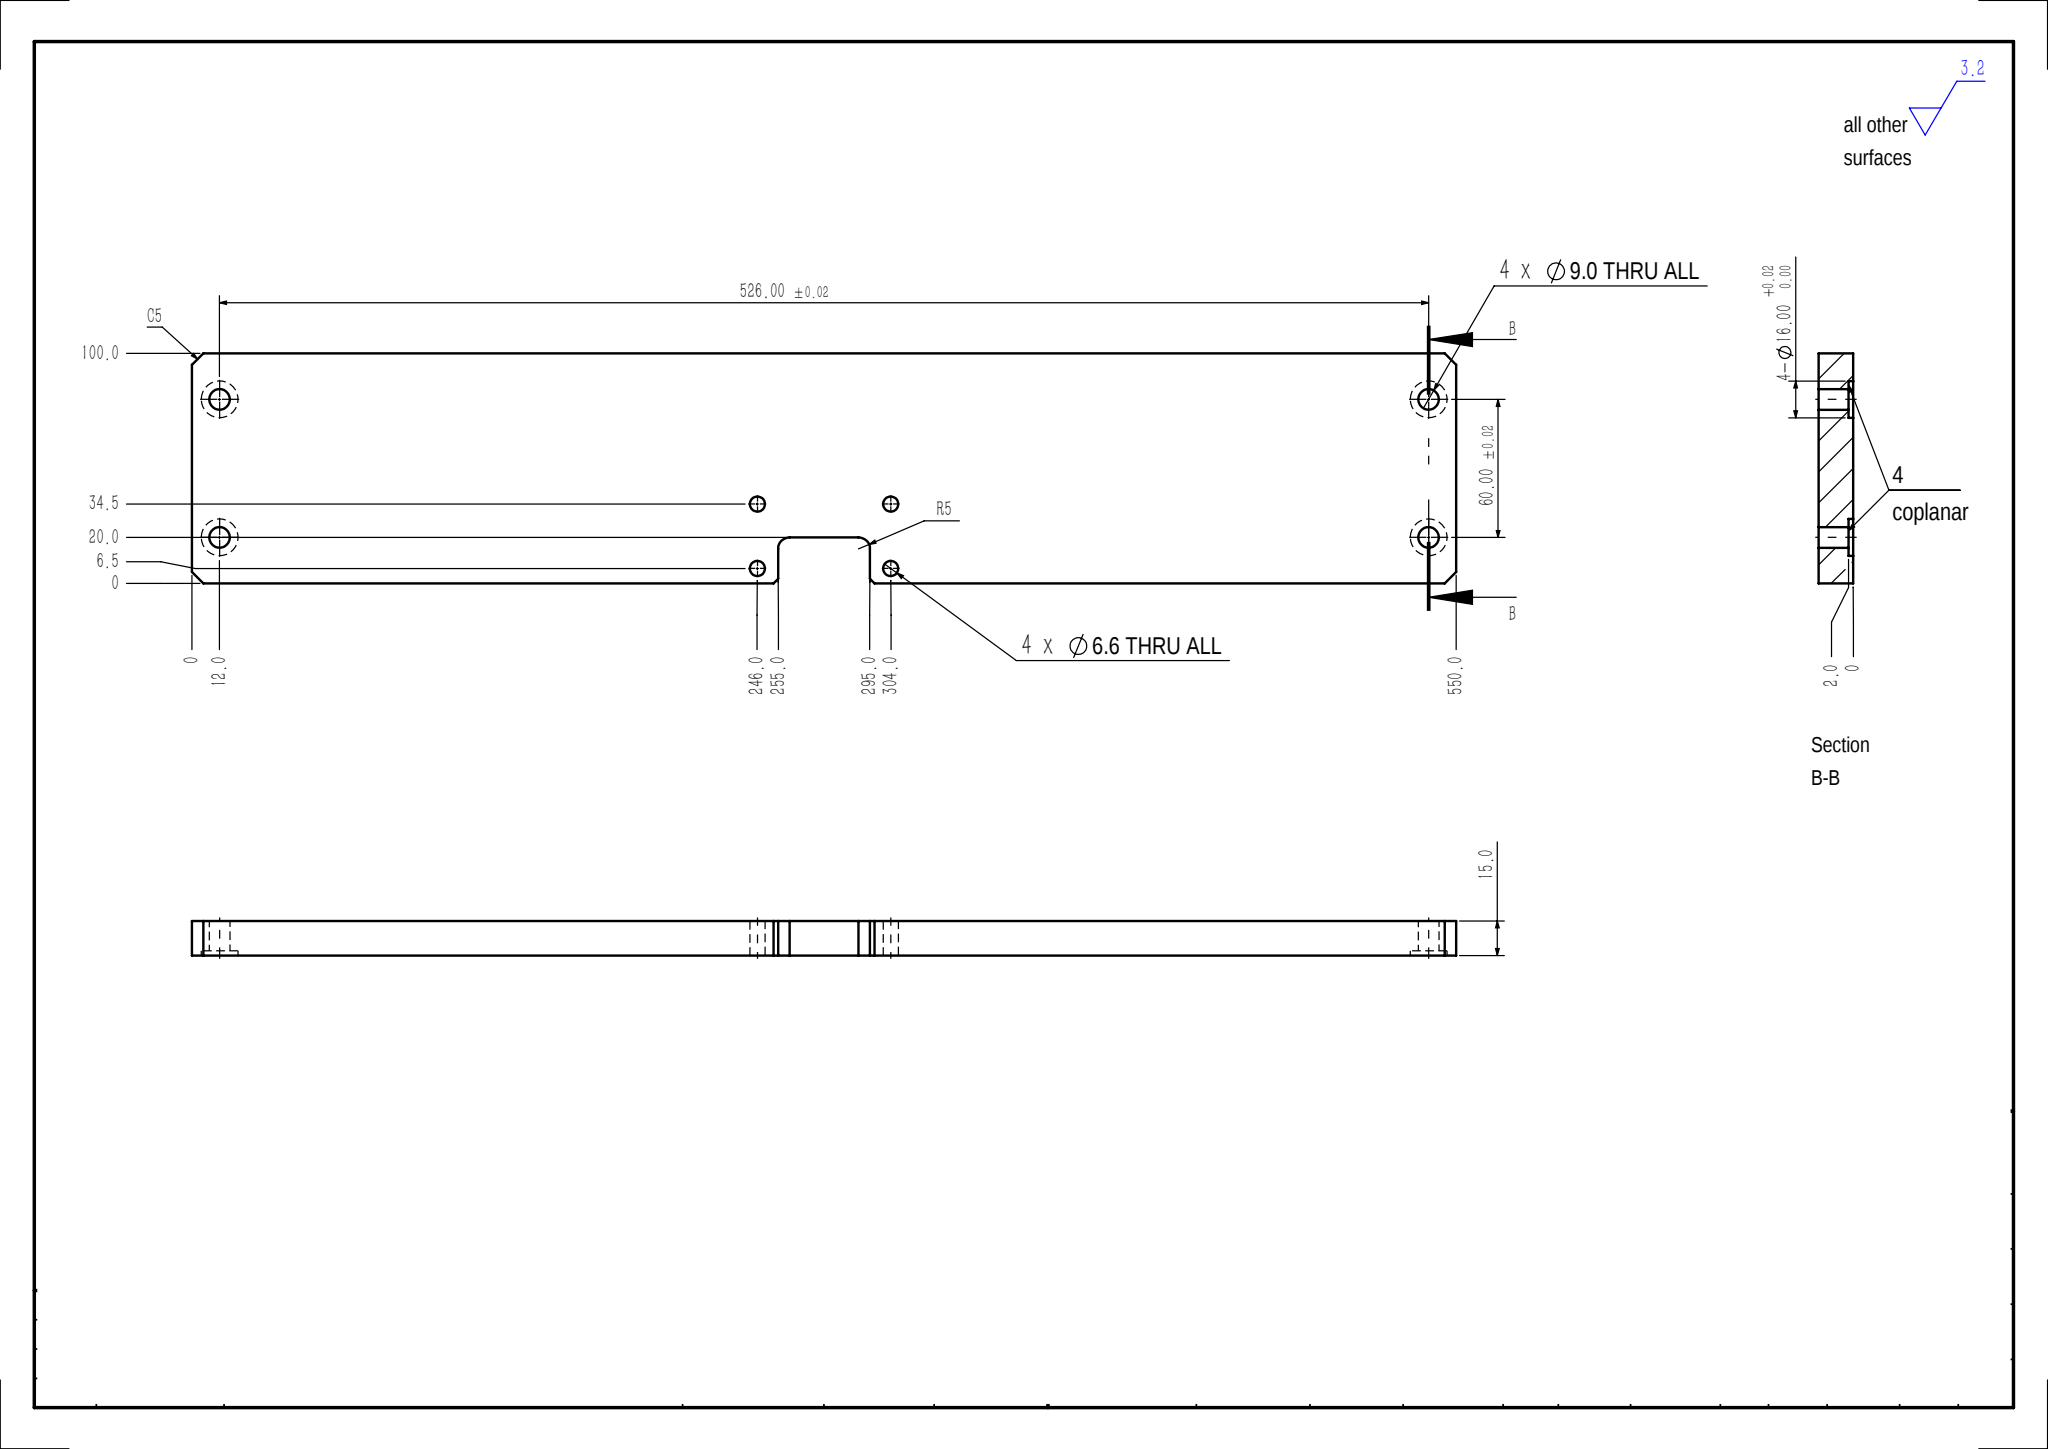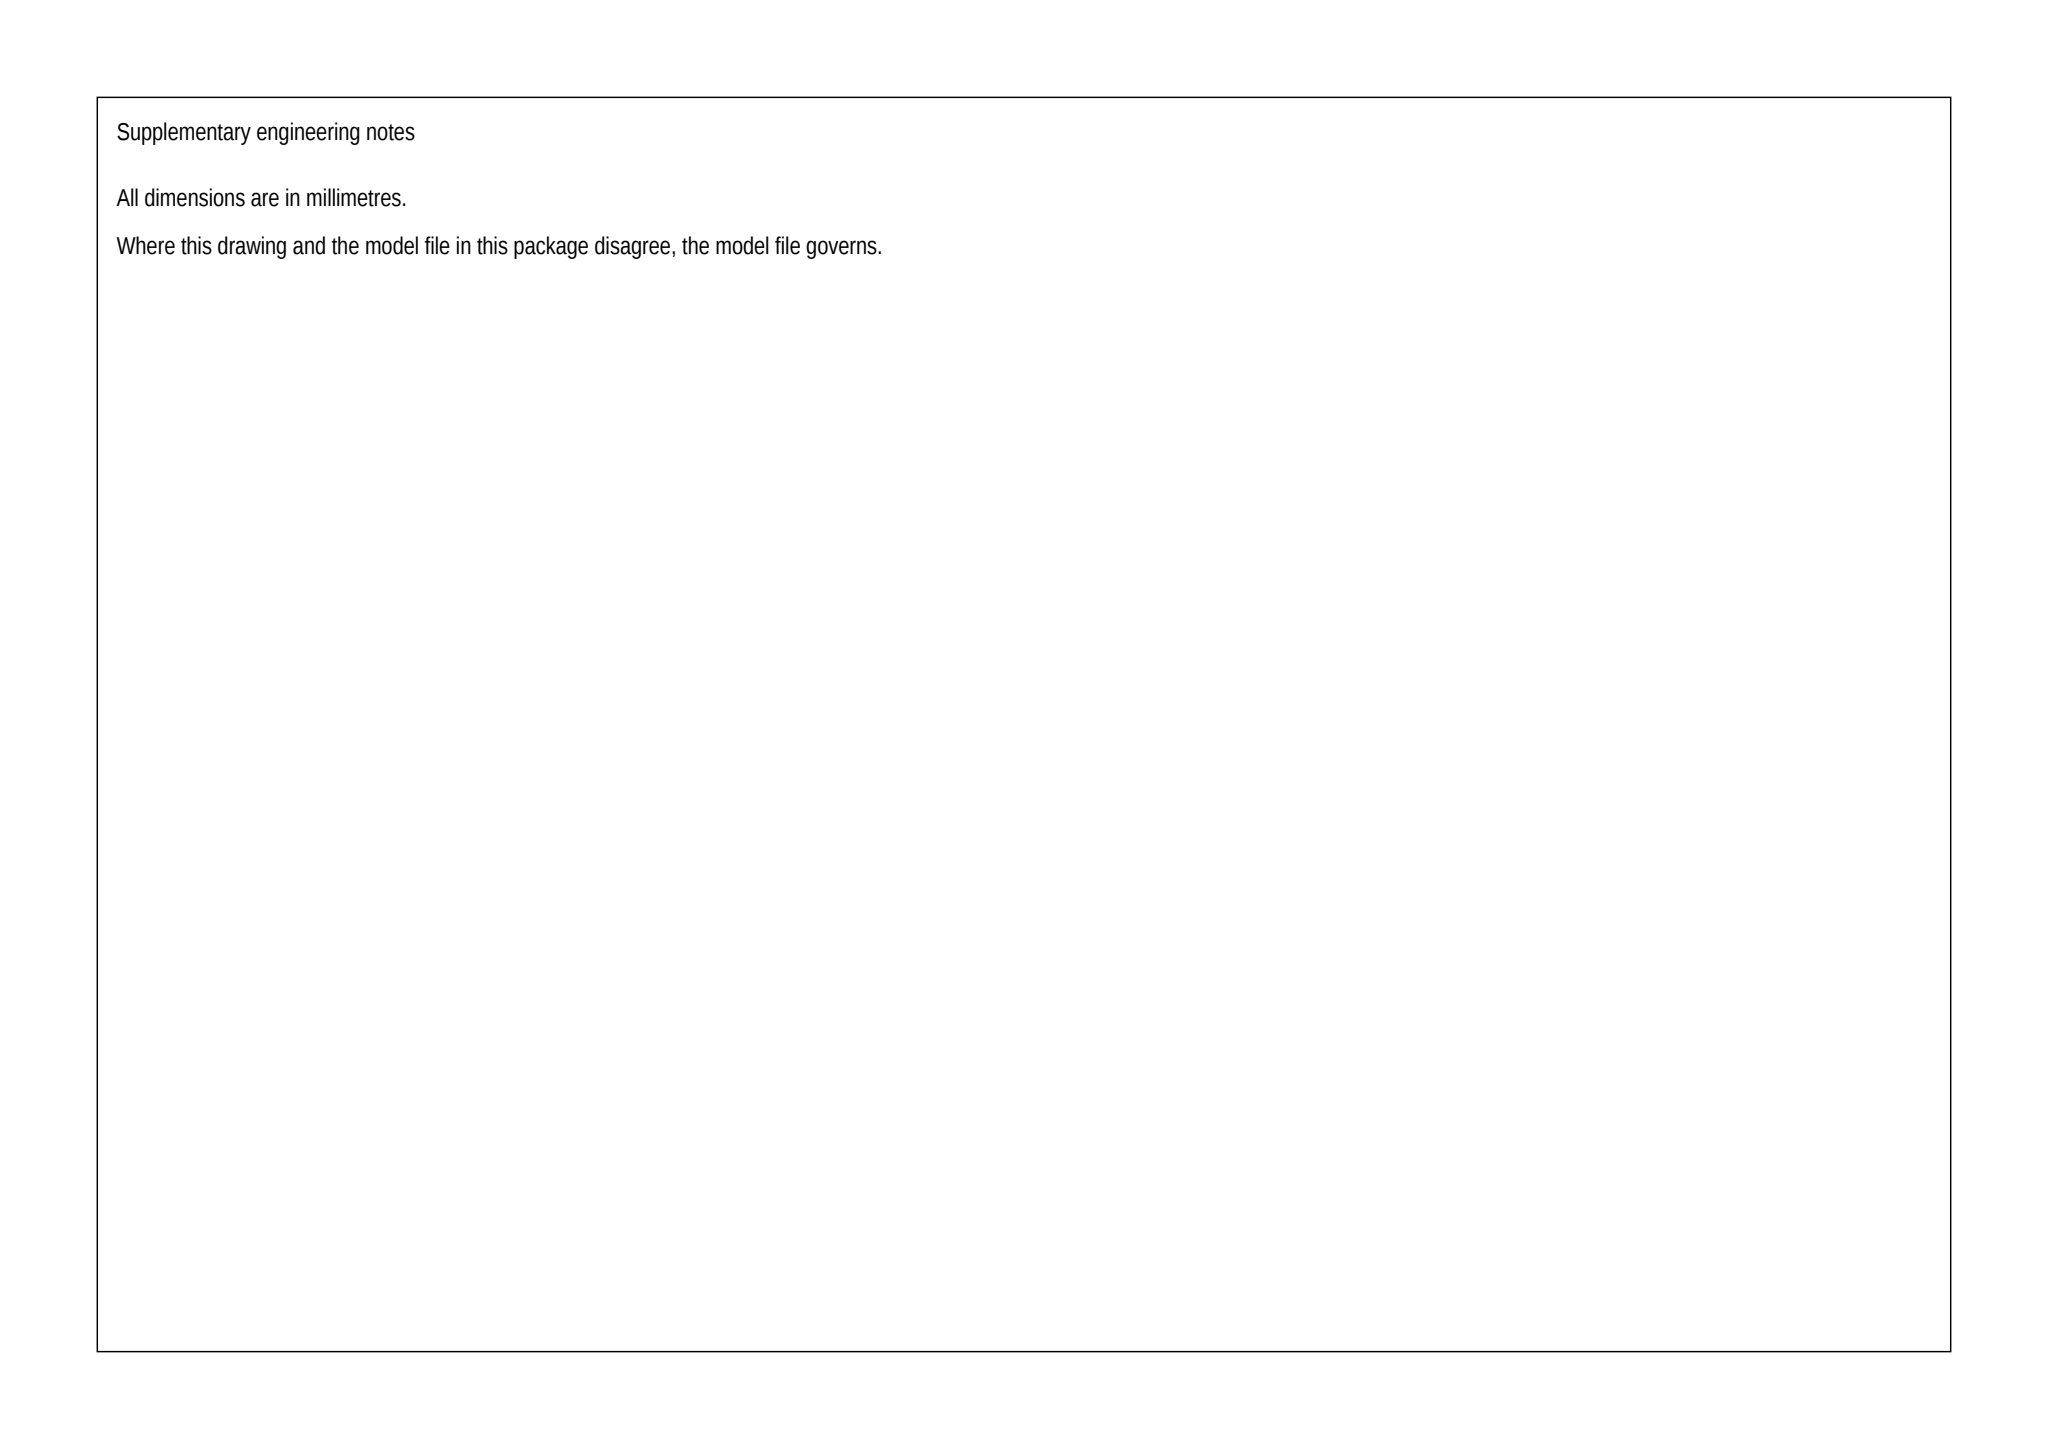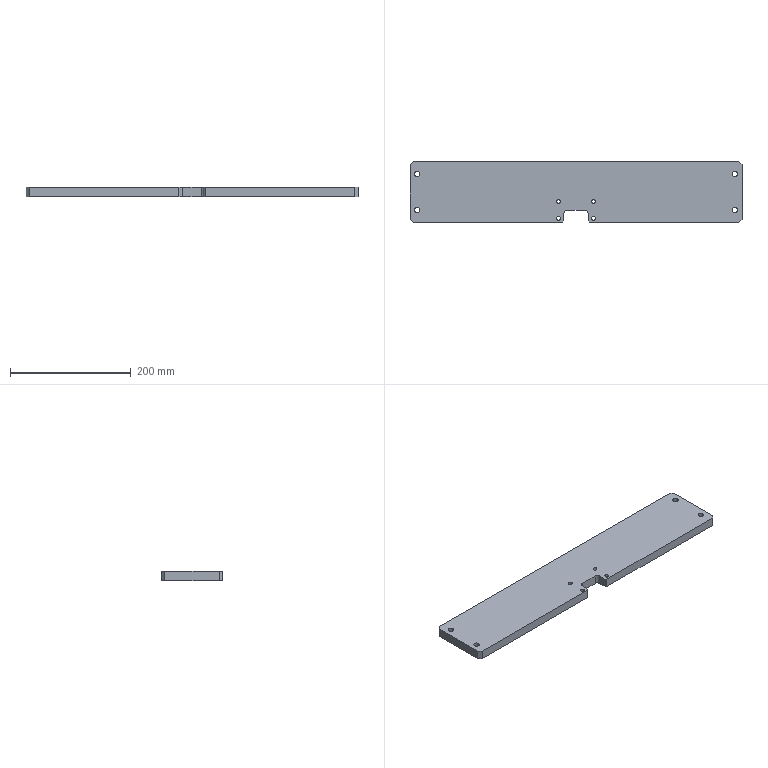Part | SolidWorks | mm | 1 solid | 46 faces | box 550 x 100 x 15 mm | volume 805382 mm3 | cylinder 26 | plane 20 | commonest cylinder face diameters 6.6 x8 16 x8 9 x8 10 x2
build123d program:
from build123d import *

# Parameters (mm, degrees)
SKETCH1_W             = 550
SKETCH1_H             = 100
BOSS_EXTRUDE1_DEPTH   = 15
M8_CLEARANCE_HOLE_1_D = 9
SKETCH5_R             = 8
CUT_EXTRUDE1_DEPTH    = 2
CHAMFER1_SIZE         = 5
SKETCH6_W             = 40
SKETCH6_H             = 20
CUT_EXTRUDE2_DEPTH    = 280.911
FILLET1_R             = 5
CHAMFER2_SIZE         = 2
M6_CLEARANCE_HOLE_1_D = 6.6


with BuildPart() as part:
    # Sketch1 → Boss-Extrude1 (new body)
    with BuildSketch(Plane.XY):
        Rectangle(SKETCH1_W, SKETCH1_H)
    extrude(amount=BOSS_EXTRUDE1_DEPTH)

    # M8 Clearance Hole 1 (through all)
    with Locations(Plane.XY.offset(15)):
        with Locations((-263, 30), (-263, -30), (263, -30), (263, 30)):
            Hole(M8_CLEARANCE_HOLE_1_D / 2)

    # Sketch5 → Cut-Extrude1 (cut)
    with BuildSketch(Plane(origin=(0, 0, 0), x_dir=(-1, 0, 0), z_dir=(0, 0, -1))):
        with Locations((-263, 30)):
            Circle(SKETCH5_R)
        with Locations((-263, -30)):
            Circle(SKETCH5_R)
        with Locations((263, -30)):
            Circle(SKETCH5_R)
        with Locations((263, 30)):
            Circle(SKETCH5_R)
    extrude(amount=-CUT_EXTRUDE1_DEPTH, mode=Mode.SUBTRACT)

    # Chamfer1
    chamfer1_edges = [part.edges().sort_by_distance(p)[0] for p in [
        (275, -50, 7.5),
        (-275, -50, 7.5),
        (-275, 50, 7.5),
        (275, 50, 7.5),
    ]]
    chamfer(chamfer1_edges, length=CHAMFER1_SIZE)

    # Sketch6 → Cut-Extrude2 (cut, through all)
    with BuildSketch(Plane(origin=(0, 0, 0), x_dir=(-1, 0, 0), z_dir=(0, 0, -1))):
        with Locations((0, -40)):
            Rectangle(SKETCH6_W, SKETCH6_H)
    extrude(amount=-CUT_EXTRUDE2_DEPTH, mode=Mode.SUBTRACT)

    # Fillet1
    fillet1_edges = [part.edges().sort_by_distance(p)[0] for p in [
        (20, -30, 7.5),
        (-20, -30, 7.5),
    ]]
    fillet(fillet1_edges, radius=FILLET1_R)

    # Chamfer2
    chamfer2_edges = [part.edges().sort_by_distance(p)[0] for p in [
        (20, -50, 7.5),
        (-20, -50, 7.5),
    ]]
    chamfer(chamfer2_edges, length=CHAMFER2_SIZE)

    # M6 Clearance Hole 1 (through all)
    with Locations(Plane(origin=(0, 0, 0), x_dir=(-1, 0, 0), z_dir=(0, 0, -1))):
        with Locations((29, -15.5), (29, -43.5), (-29, -15.5), (-29, -43.5)):
            Hole(M6_CLEARANCE_HOLE_1_D / 2)


solid = part.part